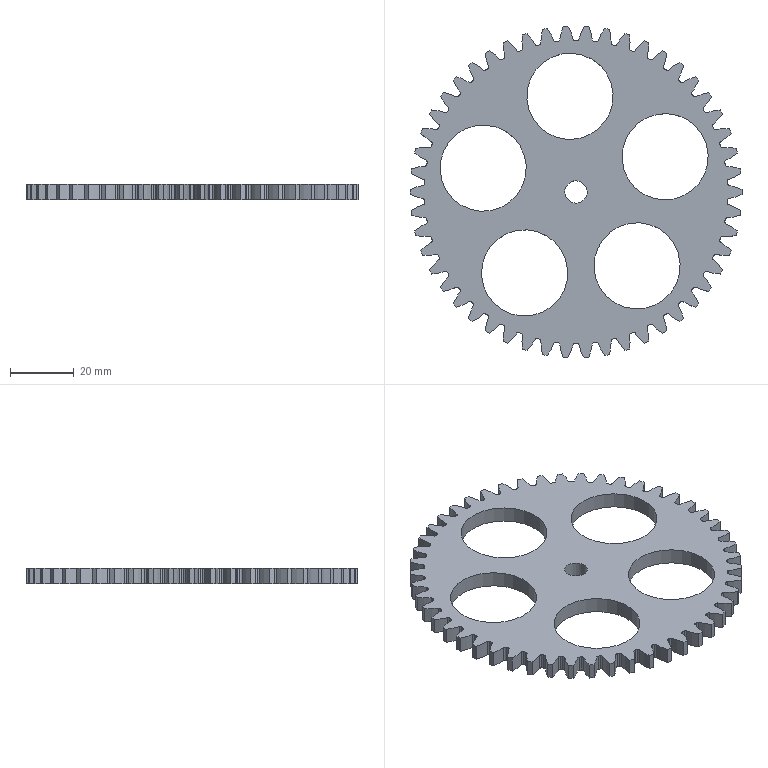Component | NX | GEAR | 1 solid | 308 faces | volume 24463 mm3 | spline 250 | cylinder 56 | plane 2 | commonest cylinder face diameters 94.95 x50 27 x5 7 x1